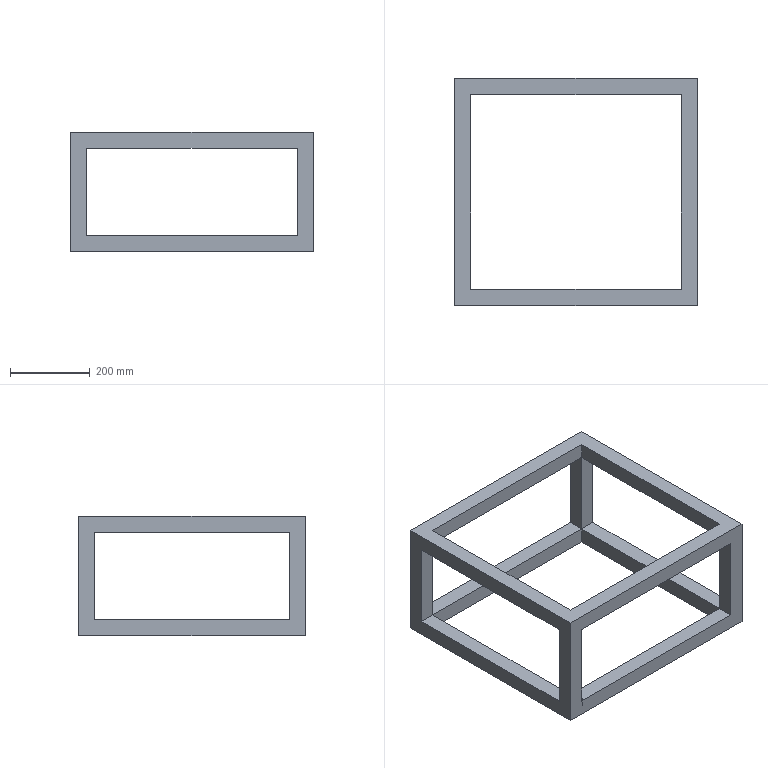Component | SolidWorks | AssemblyVibratoryFeederChassis-1_Frame01-1-1 | 1 solid | 48 faces | box 610 x 570 x 300 mm | volume 8420190 mm3 | plane 30 | cylinder 10 | cone 8 | commonest cylinder face diameters 16 x8 5 x2
build123d program:
from build123d import *

# Parameters (mm, degrees)
SKETCH1_W              = 610
SKETCH1_H              = 300
EXTRUDE1_DEPTH         = 570
SKETCH2_W              = 530
SKETCH2_H              = 220
EXTRUDE2_DEPTH         = 664.645
SKETCH3_W              = 490
SKETCH3_H              = 220
EXTRUDE3_DEPTH         = 849.233
SKETCH4_W              = 530
SKETCH4_H              = 490
EXTRUDE4_DEPTH         = 660
M16_TAPPED_HOLE1_D     = 16
M16_TAPPED_HOLE1_DEPTH = 32
M16_TAPPED_HOLE1_TIP   = 4.807
SKETCH8_R              = 2.5
CUT_EXTRUDE1_DEPTH     = 60


with BuildPart() as part:
    # Sketch1 → Extrude1 (new body)
    with BuildSketch(Plane.XY):
        Rectangle(SKETCH1_W, SKETCH1_H)
    extrude(amount=-EXTRUDE1_DEPTH)

    # Sketch2 → Extrude2 (cut, through all)
    with BuildSketch(Plane.XY):
        Rectangle(SKETCH2_W, SKETCH2_H)
    extrude(amount=-EXTRUDE2_DEPTH, mode=Mode.SUBTRACT)

    # Sketch3 → Extrude3 (cut, through all)
    with BuildSketch(Plane(origin=(305, 0, 0), x_dir=(0, 0, -1), z_dir=(1, 0, 0))):
        with Locations((285, 0)):
            Rectangle(SKETCH3_W, SKETCH3_H)
    extrude(amount=-EXTRUDE3_DEPTH, mode=Mode.SUBTRACT)

    # Sketch4 → Extrude4 (cut)
    with BuildSketch(Plane(origin=(0, 150, 0), x_dir=(1, 0, 0), z_dir=(0, 1, 0))):
        with Locations((0, 285)):
            Rectangle(SKETCH4_W, SKETCH4_H)
    extrude(amount=-EXTRUDE4_DEPTH, mode=Mode.SUBTRACT)

    # M16 Tapped Hole1
    with Locations(Plane.XZ.offset(150)):
        with Locations((-285, -20), (-285, -550), (285, -550), (285, -20)):
            Hole(M16_TAPPED_HOLE1_D / 2, depth=M16_TAPPED_HOLE1_DEPTH)
            with Locations((0, 0, -(M16_TAPPED_HOLE1_DEPTH + M16_TAPPED_HOLE1_TIP / 2))):  # 118° drill point
                Cone(0, M16_TAPPED_HOLE1_D / 2, M16_TAPPED_HOLE1_TIP, mode=Mode.SUBTRACT)

    # Sketch8 → Cut-Extrude1 (cut)
    with BuildSketch(Plane.XZ.offset(150)):
        with Locations(Location((-260, -5, 0), (0, 0, 270))):
            Circle(SKETCH8_R)
    extrude(amount=-CUT_EXTRUDE1_DEPTH, mode=Mode.SUBTRACT)


solid = part.part

# Placed as in the assembly
solid = solid.moved(Location((-102.449, -301.176, 78), (90, 0, 0)))